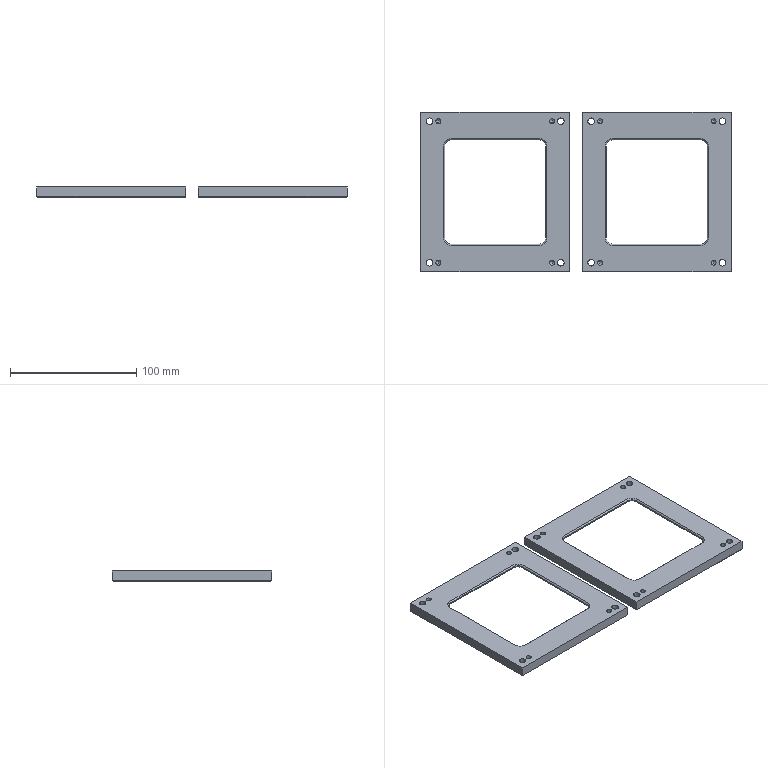CAM job | Mastercam | mm | 14 operations | part box 246 x 126 x 8
1. Facing | 24 - 100 平铣刀
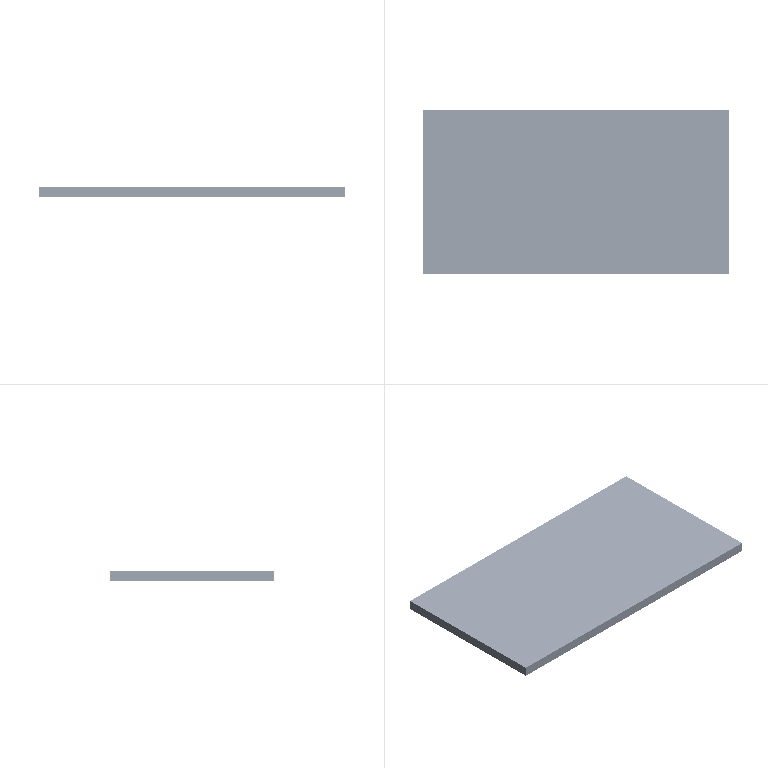2. 2D High Speed (2D Area Mill) | 10 - 10 平铣刀
3. Contour (2D) | 10 - 10 平铣刀
4. Contour (Ramp) | 4 - 4 平铣刀
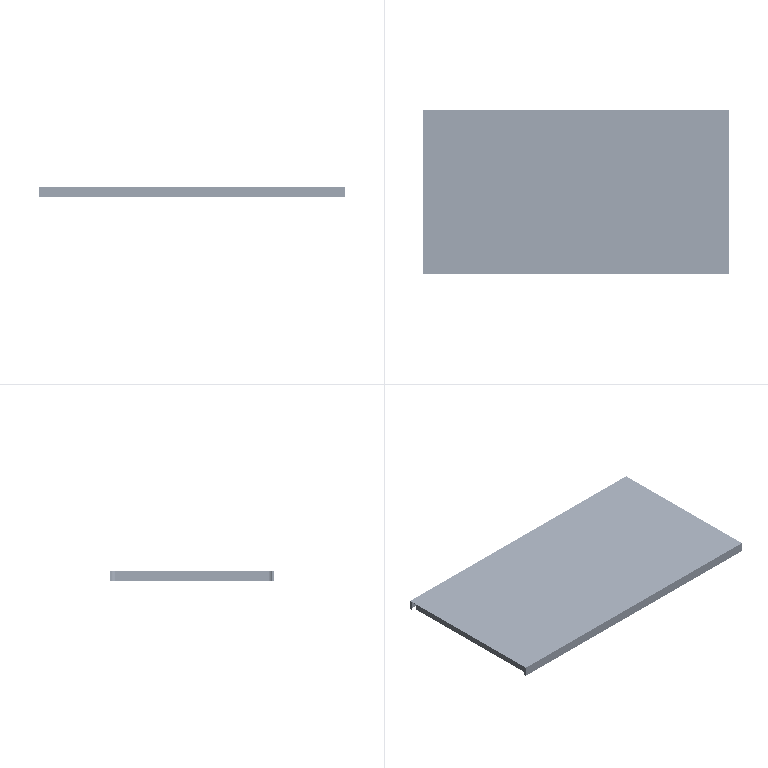5. Contour (Ramp) | 4 - 4 平铣刀
6. Contour (2D chamfer) | 7 - 4 倒角刀
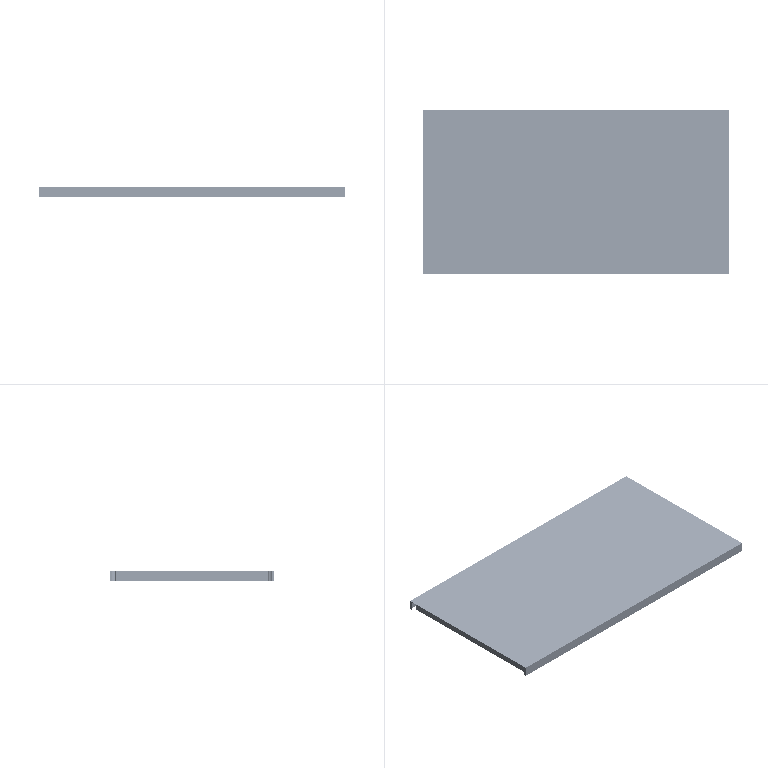7. Contour (2D chamfer) | 7 - 4 倒角刀
8. Drill/Counterbore | 7 - 4 倒角刀
9. Contour (Ramp) | 3 - 3 平铣刀
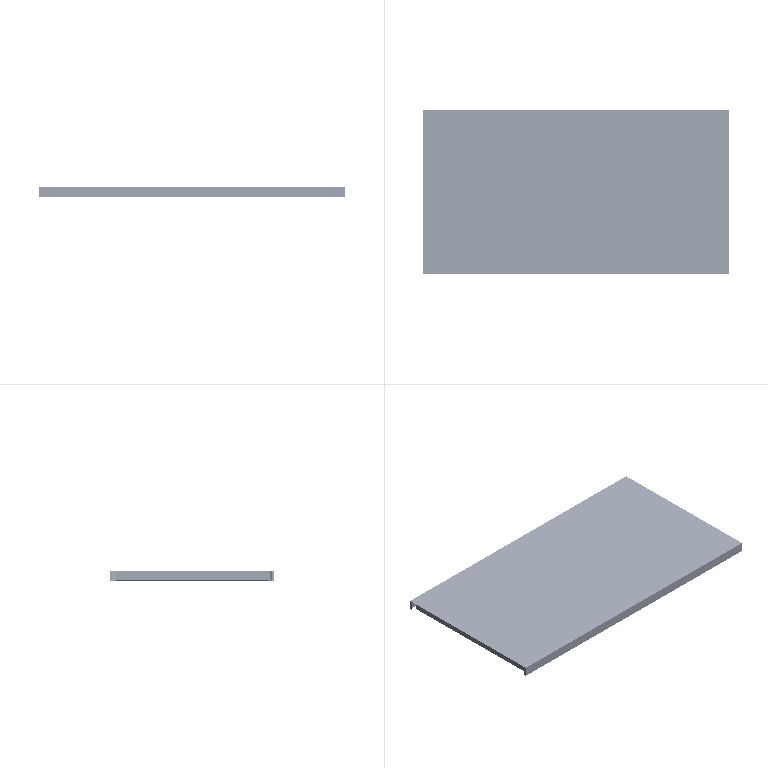10. Contour (Ramp) | 3 - 3 平铣刀
11. Contour (2D chamfer) | 7 - 4 倒角刀
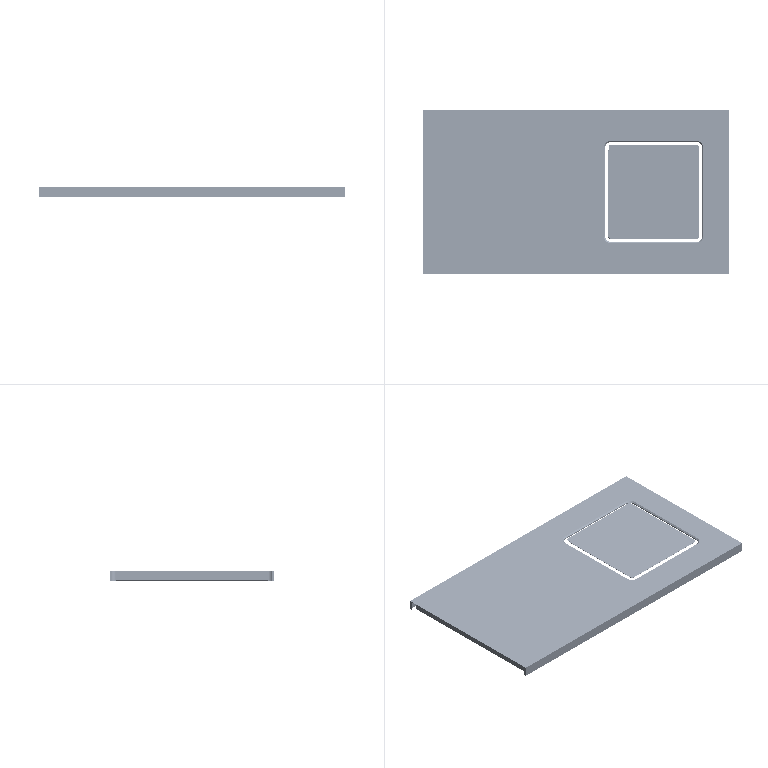12. Drill/Counterbore | 7 - 4 倒角刀
13. Contour (2D chamfer) | 7 - 4 倒角刀
14. Contour (2D) | 10 - 10 平铣刀